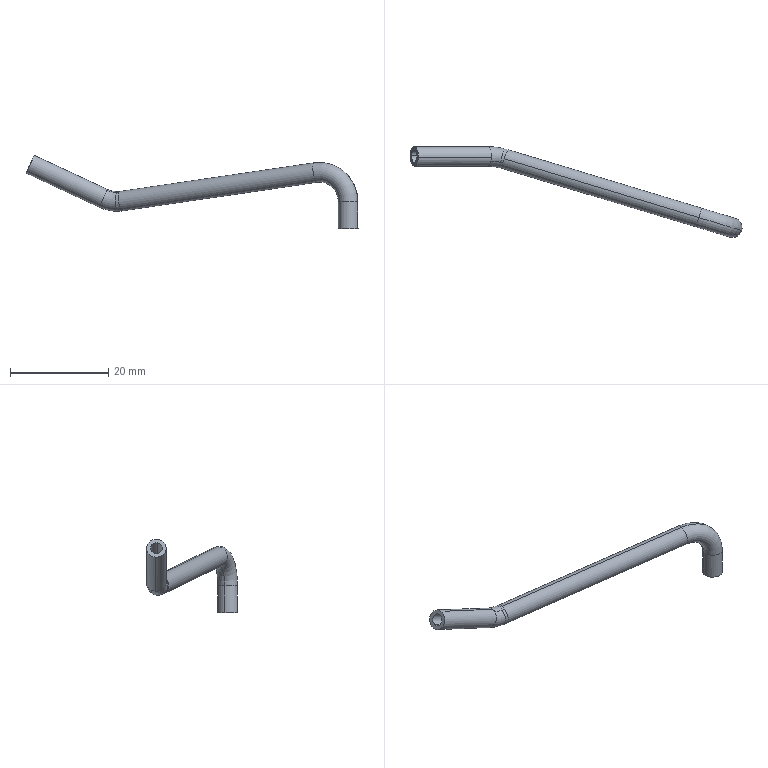Component | SolidWorks | WaterPipe4-1 | 1 solid | 26 faces | box 67.55 x 18.5 x 14.89 mm | volume 625 mm3 | torus 12 | cylinder 12 | plane 2 | commonest cylinder face diameters 2.4 x6 4 x6
build123d program:
from build123d import *

# Parameters (mm, degrees)
SCAN_THIN_FEATURE1_PROFILE_R   = 2
SCAN_THIN_FEATURE1_PROFILE_R_2 = 1.2


with BuildPart() as part:
    # Scan-Thin Feature1: sweep along a curve in space
    with BuildLine() as scan_thin_feature1_path:
        Line((0, 0, 15), (0, 0, 9.534))
        ThreePointArc((6.837, 0.0849, 3.593), (2.064, 0.02564, 5.005), (0, 0, 9.534))
        Line((6.837, 0.0849, 3.593), (48.188, 0.5985, 9.419))
        ThreePointArc((51.908, 0.121, 8.854), (50.106, 0.4879, 9.41), (48.188, 0.5985, 9.419))
        Line((51.908, 0.121, 8.854), (66.19, -3.998, 1.922))
    # Scan-Thin Feature1 profile (on start of the path) → Scan-Thin Feature1 (sweep)
    with BuildSketch(Plane(origin=(0, 0, 15), x_dir=(-1, 0, 0), z_dir=(0, 0, -1))):
        Circle(SCAN_THIN_FEATURE1_PROFILE_R)
        Circle(SCAN_THIN_FEATURE1_PROFILE_R_2, mode=Mode.SUBTRACT)
    sweep(path=scan_thin_feature1_path.line)


solid = part.part

# Placed as in the assembly
solid = solid.moved(Location((-5.981, 20.506, 193.534), (-180, 0, -163.913)))